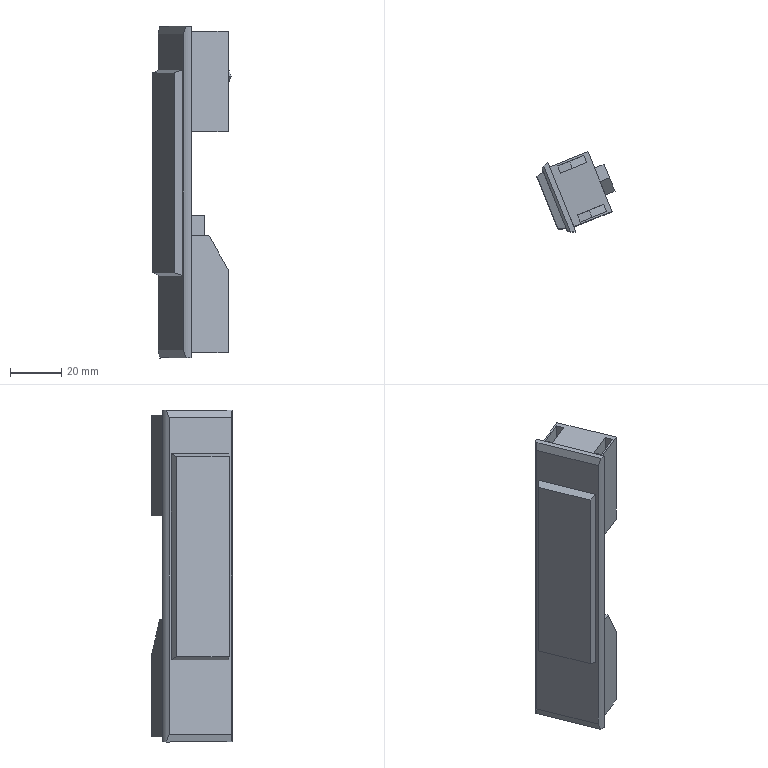Component | SolidWorks | RightDoorAssembly-1_LinkRodLock-1_Lock-1_LockBody-1 | 1 solid | 48 faces | box 30.31 x 31.12 x 129 mm | volume 46975 mm3 | plane 42 | cylinder 6 | commonest cylinder face diameters 5 x2 6 x2 13.843 x2
build123d program:
from build123d import *

# Parameters (mm, degrees)
SKETCH1_W           = 32
SKETCH1_H           = 129
EXTRUDE1_DEPTH      = 1.5
CUT_EXTRUDE2_DEPTH  = 130.997
CUT_EXTRUDE3_DEPTH  = 25
SKETCH5_W           = 25
SKETCH5_H           = 39
EXTRUDE2_DEPTH      = 16
EXTRUDE3_DEPTH      = 4
SKETCH8_R           = 3
CUT_EXTRUDE4_DEPTH  = 5
SKETCH9_W           = 25
SKETCH9_H           = 45.5
EXTRUDE4_DEPTH      = 16
CUT_EXTRUDE5_DEPTH  = 15
SKETCH16_W          = 16
SKETCH16_H          = 8
BOSS_EXTRUDE1_DEPTH = 8
SKETCH17_R          = 2.5
CUT_EXTRUDE9_DEPTH  = 10
SKETCH18_W          = 3
SKETCH18_H          = 11
CUT_EXTRUDE10_DEPTH = 71.5
SKETCH12_W          = 24
SKETCH12_H          = 80
EXTRUDE5_DEPTH      = 3
EXTRUDE5_TAPER      = 20


with BuildPart() as part:
    # Sketch1 → Extrude1 (new, symmetric)
    with BuildSketch(Plane.XY):
        Rectangle(SKETCH1_W, SKETCH1_H)
    extrude(amount=EXTRUDE1_DEPTH, both=True)

    # Sketch2 → Cut-Extrude2 (cut, symmetric)
    with BuildSketch(Plane.XZ.offset(64.5)):
        with BuildLine():
            Line((-33.384, -55.642), (13, -1.5))
            ThreePointArc((13, -1.5), (13.934, -0.09223), (14.5, 1.5))
            Line((14.5, 1.5), (29.984, 71.093))
            Line((29.984, 71.093), (157.519, 7.325))
            Line((157.519, 7.325), (94.151, -119.41))
            Line((94.151, -119.41), (-33.384, -55.642))
        make_face()
    cut_extrude2 = extrude(amount=CUT_EXTRUDE2_DEPTH, both=True, mode=Mode.SUBTRACT)

    # Mirror1: Cut-Extrude2 across plane
    add(cut_extrude2.mirror(Plane(origin=(0, 0, 0), x_dir=(0, 0, 1), z_dir=(1, 0, 0))), mode=Mode.SUBTRACT)

    # Sketch4 → Cut-Extrude3 (cut, symmetric)
    with BuildSketch(Plane(origin=(0, 0, 0), x_dir=(0, 0, -1), z_dir=(1, 0, 0))):
        Polygon((0.5, 64.5), (1.5, 64.5), (1.5, 61.5), align=None)
    cut_extrude3 = extrude(amount=CUT_EXTRUDE3_DEPTH, both=True, mode=Mode.SUBTRACT)

    # Mirror2: Cut-Extrude3 across plane
    add(cut_extrude3.mirror(Plane.ZX), mode=Mode.SUBTRACT)

    # Sketch5 → Extrude2 (add)
    with BuildSketch(Plane.XY.offset(1.5)):
        with Locations((0, 43)):
            Rectangle(SKETCH5_W, SKETCH5_H)
    extrude(amount=EXTRUDE2_DEPTH)

    # Sketch7 → Extrude3 (add)
    with BuildSketch(Plane.XY.offset(17.5)):
        Polygon((0, 50.657), (5.657, 45), (0, 39.343), (-5.657, 45), align=None)
    extrude(amount=EXTRUDE3_DEPTH)

    # Sketch8 → Cut-Extrude4 (cut)
    with BuildSketch(Plane.XY.offset(21.5)):
        with Locations((0, 45)):
            Circle(SKETCH8_R)
    extrude(amount=-CUT_EXTRUDE4_DEPTH, mode=Mode.SUBTRACT)

    # Sketch9 → Extrude4 (add)
    with BuildSketch(Plane.XY.offset(1.5)):
        with Locations((0, -39.75)):
            Rectangle(SKETCH9_W, SKETCH9_H)
    extrude(amount=EXTRUDE4_DEPTH)

    # Sketch10 → Cut-Extrude5 (cut, symmetric)
    with BuildSketch(Plane(origin=(0, 0, 0), x_dir=(0, 0, -1), z_dir=(1, 0, 0))):
        Polygon((-9.5, -17), (-17.5, -30), (-17.5, -17), align=None)
    extrude(amount=CUT_EXTRUDE5_DEPTH, both=True, mode=Mode.SUBTRACT)

    # Sketch16 → Boss-Extrude1 (add)
    with BuildSketch(Plane.XY.offset(1.5)):
        with Locations((0, -13)):
            Rectangle(SKETCH16_W, SKETCH16_H)
    extrude(amount=BOSS_EXTRUDE1_DEPTH)

    # Sketch17 → Cut-Extrude9 (cut)
    with BuildSketch(Plane.XY.offset(9.5)):
        with Locations((0, -13)):
            Circle(SKETCH17_R)
    extrude(amount=-CUT_EXTRUDE9_DEPTH, mode=Mode.SUBTRACT)

    # Sketch18 → Cut-Extrude10 (cut)
    with BuildSketch(Plane(origin=(0, 62.5, 0), x_dir=(1, 0, 0), z_dir=(0, 1, 0))):
        with Locations((10.25, -10)):
            Rectangle(SKETCH18_W, SKETCH18_H)
        with Locations((-10.25, -10)):
            Rectangle(SKETCH18_W, SKETCH18_H)
    extrude(amount=-CUT_EXTRUDE10_DEPTH, mode=Mode.SUBTRACT)

    # Sketch12 → Extrude5 (add)
    with BuildSketch(Plane(origin=(0, 0, -1.5), x_dir=(-1, 0, 0), z_dir=(0, 0, -1))):
        with Locations((0, 7.5)):
            Rectangle(SKETCH12_W, SKETCH12_H)
    extrude(amount=EXTRUDE5_DEPTH, taper=EXTRUDE5_TAPER)


solid = part.part

# Placed as in the assembly
solid = solid.moved(Location((-335.608, 398.631, 896.2), (-90, 68.015, -180)))